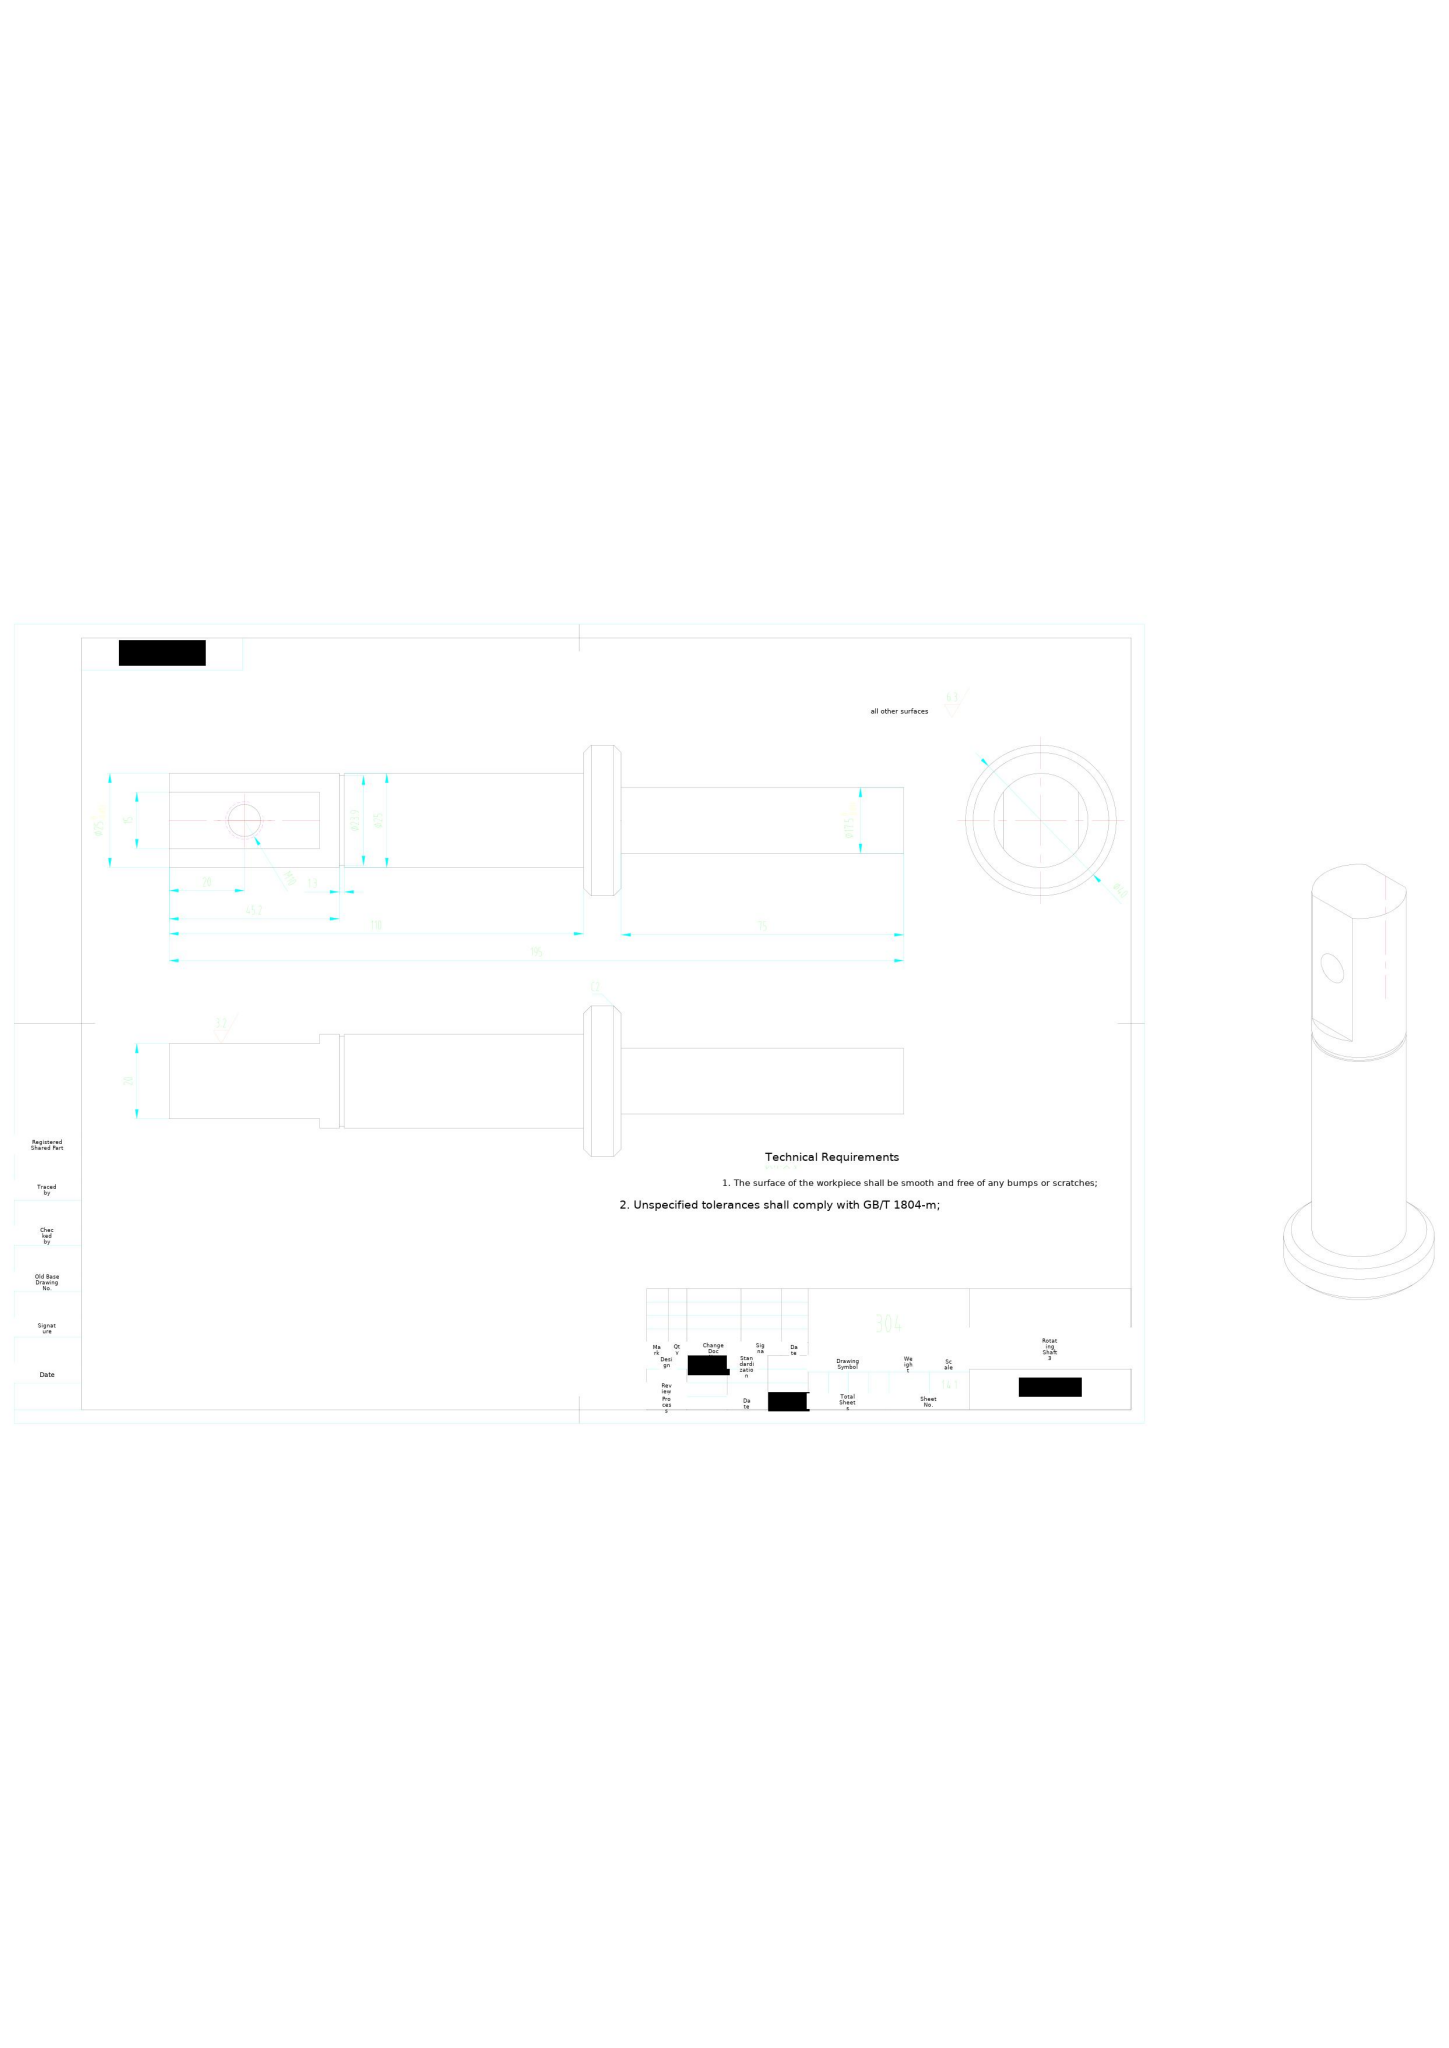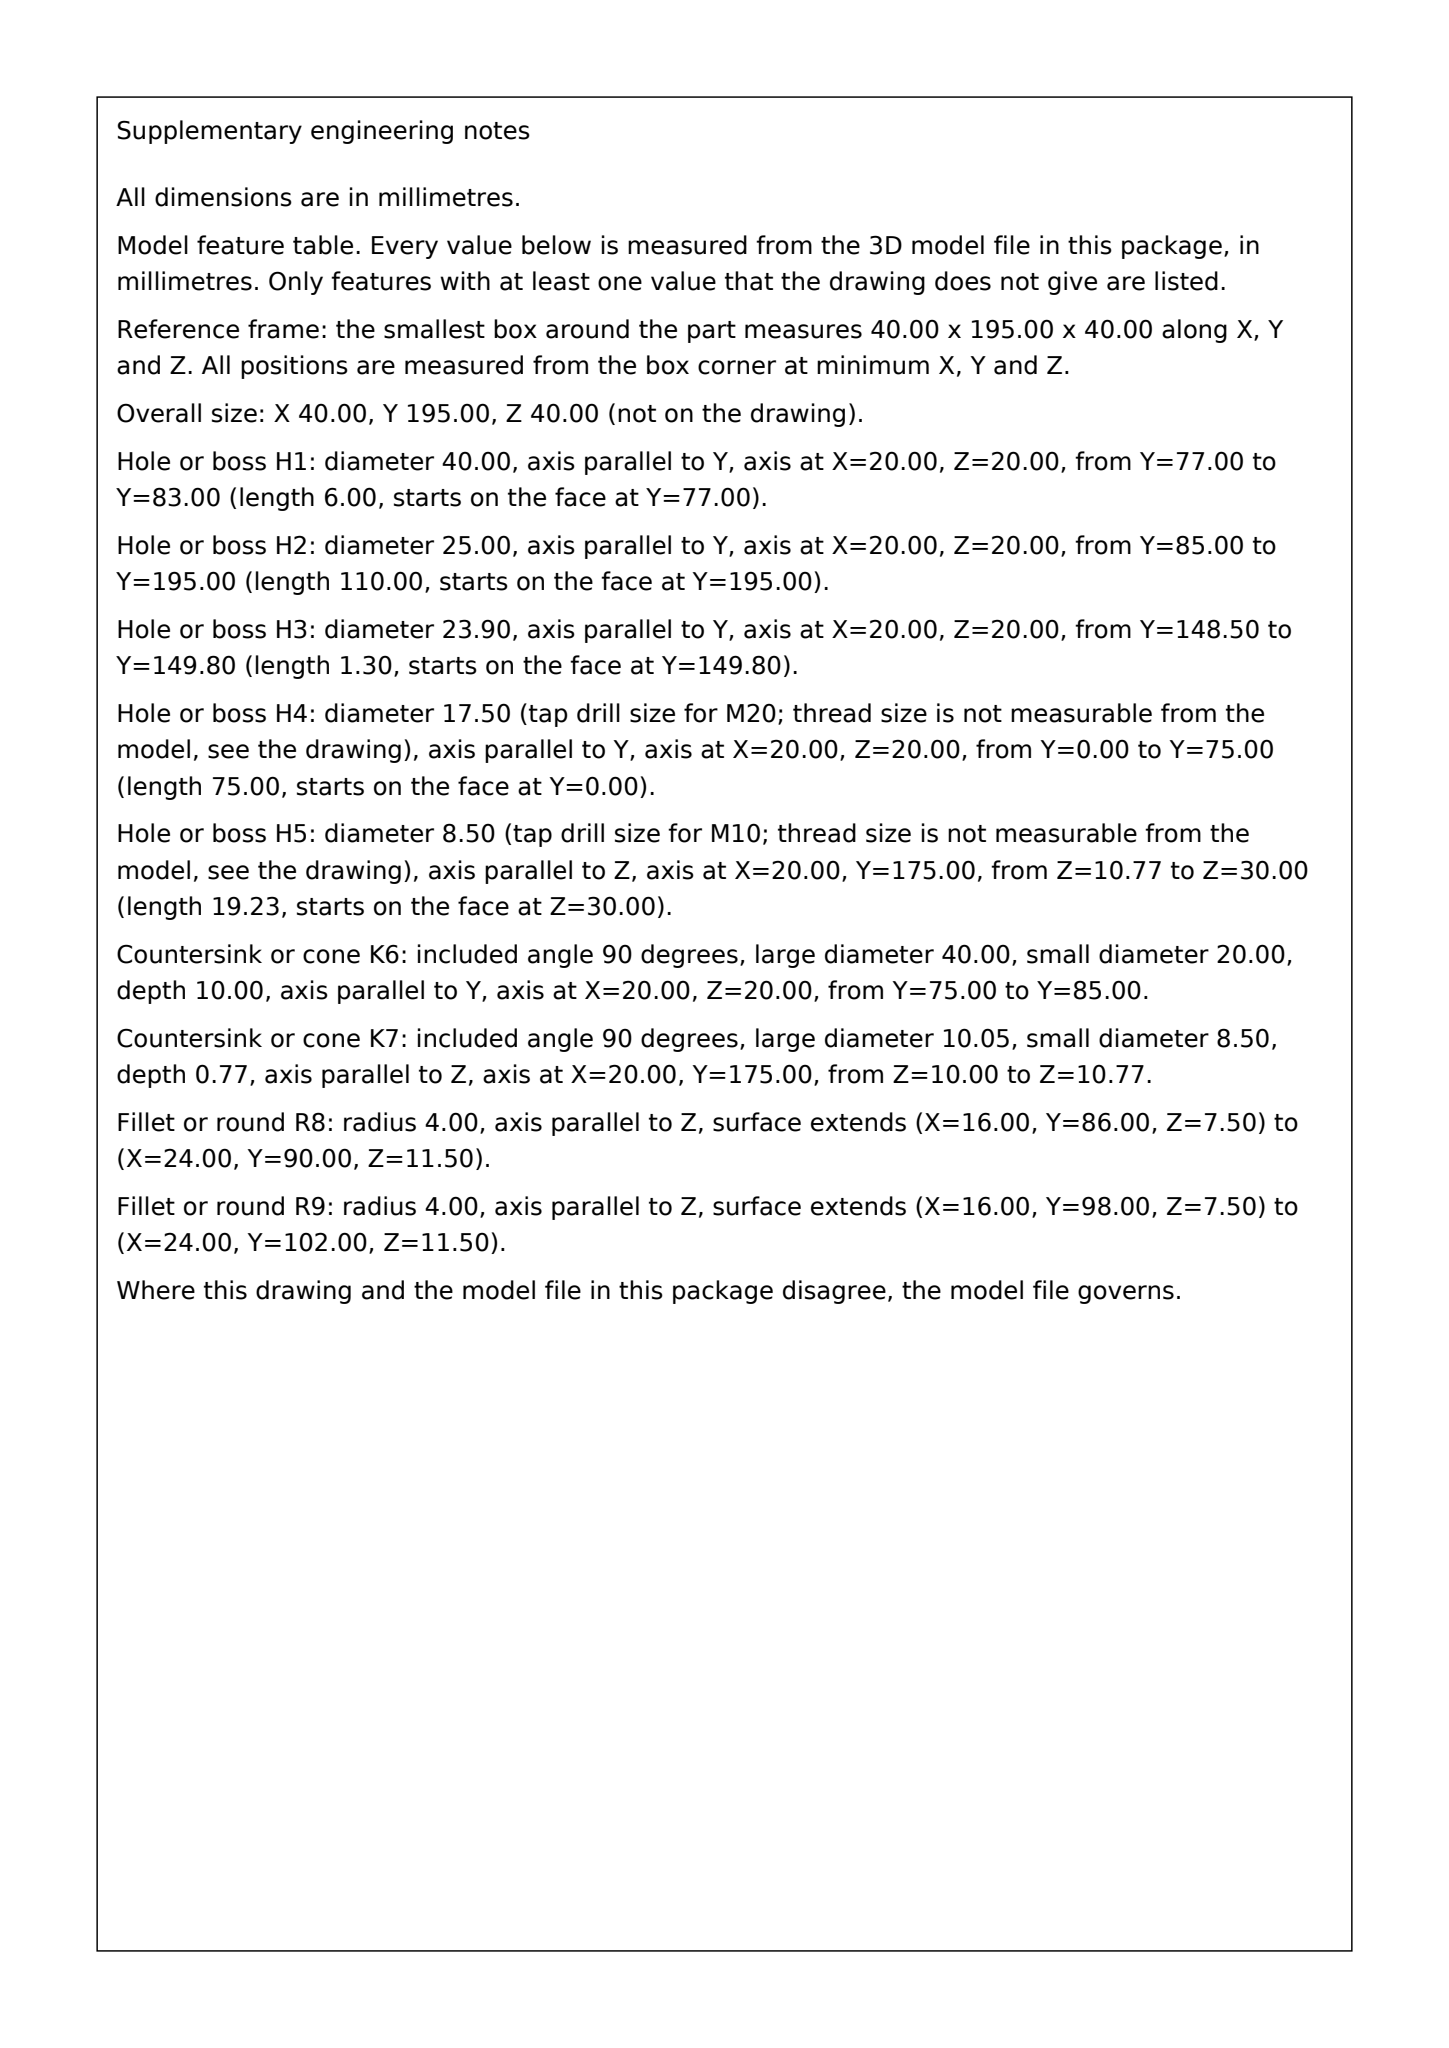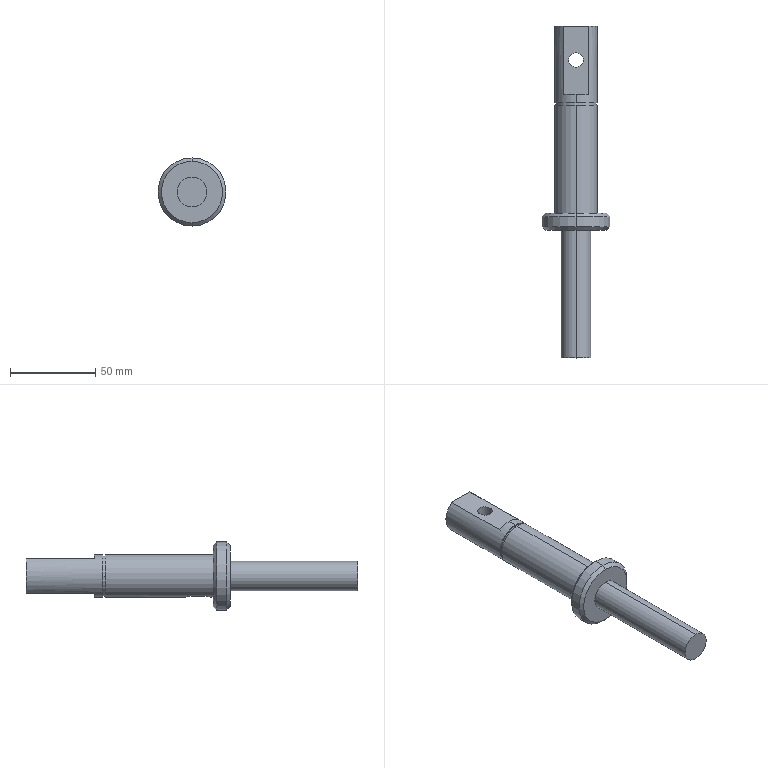Part | SolidWorks | mm | material 304 | 1 solid | 33 faces | box 40 x 195 x 40 mm | volume 80439 mm3 | cylinder 14 | plane 13 | cone 6 | commonest cylinder face diameters 25 x4 17.5 x2 8.5 x2 23.9 x2 40 x2 8 x2